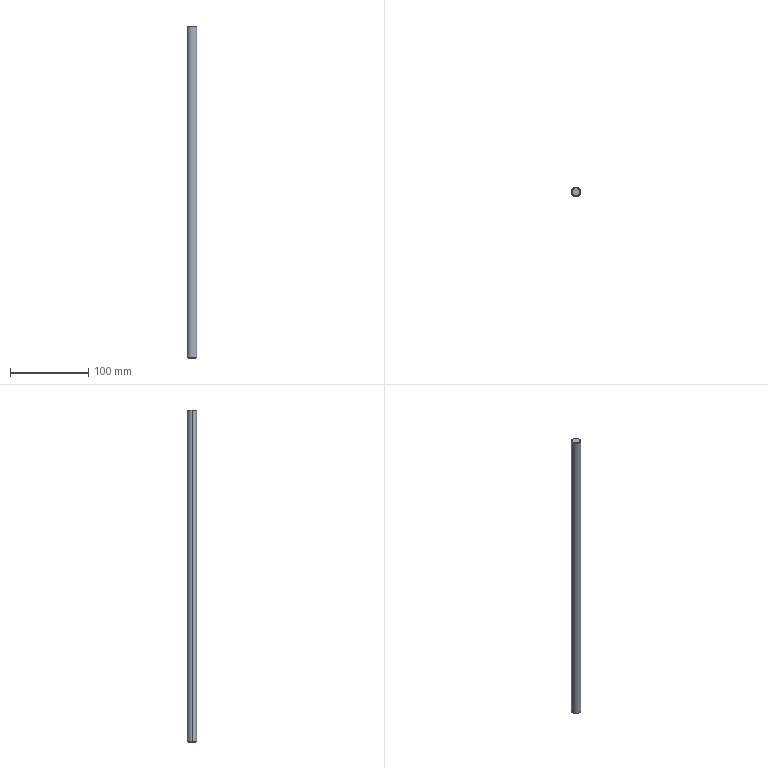Component | SolidWorks | 50-2 | 1 solid | 8 faces | box 12 x 12 x 425 mm | volume 48031 mm3 | cone 4 | cylinder 2 | plane 2 | commonest cylinder face diameters 12 x2
build123d program:
from build123d import *

# Parameters (mm, degrees)
SKETCH1_W     = 425
SKETCH1_H     = 6
CHAMFER1_SIZE = 1


with BuildPart() as part:
    # Sketch1 → Revolve1 (revolve)
    with BuildSketch(Plane.XY, mode=Mode.PRIVATE) as revolve1_sk:
        with Locations((212.5, 3)):
            Rectangle(SKETCH1_W, SKETCH1_H)
    revolve(revolve1_sk.sketch.rotate(Axis((0, 0, 0), (1, 0, 0)), 90), axis=Axis((0, 0, 0), (1, 0, 0)))

    # Chamfer1
    chamfer1_edges = [part.edges().sort_by_distance(p)[0] for p in [
        (425, 0, -6),
        (0, 0, -6),
    ]]
    chamfer(chamfer1_edges, length=CHAMFER1_SIZE)


solid = part.part

# Placed as in the assembly
solid = solid.moved(Location((0, -38, 427.5), (0, 90, 0)))
STEP:
#1=COLOUR_RGB('',0.7922,0.8196,0.9333);
#2=FILL_AREA_STYLE_COLOUR('',#1);
#3=FILL_AREA_STYLE('',(#2));
#4=SURFACE_STYLE_FILL_AREA(#3);
#5=SURFACE_SIDE_STYLE('',(#4));
#6=SURFACE_STYLE_USAGE(.BOTH.,#5);
#7=PRESENTATION_STYLE_ASSIGNMENT((#6));
#8=CARTESIAN_POINT('',(0.1969,-1.496,16.831));
#9=VERTEX_POINT('',#8);
#10=CARTESIAN_POINT('',(-0.1969,-1.496,16.831));
#11=VERTEX_POINT('',#10);
#12=CARTESIAN_POINT('',(-0.,-1.496,16.831));
#13=DIRECTION('',(0.,0.,1.));
#14=DIRECTION('',(-1.,0.,0.));
#15=AXIS2_PLACEMENT_3D('',#12,#13,#14);
#16=CIRCLE('',#15,0.1969);
#17=EDGE_CURVE('',#9,#11,#16,.T.);
#18=ORIENTED_EDGE('',*,*,#17,.F.);
#19=CARTESIAN_POINT('',(0.2362,-1.496,16.791));
#20=VERTEX_POINT('',#19);
#21=CARTESIAN_POINT('',(0.1969,-1.496,16.831));
#22=DIRECTION('',(0.7071,-0.,-0.7071));
#23=VECTOR('',#22,39.37);
#24=LINE('',#21,#23);
#25=EDGE_CURVE('',#9,#20,#24,.T.);
#26=ORIENTED_EDGE('',*,*,#25,.T.);
#27=CARTESIAN_POINT('',(-0.2362,-1.496,16.791));
#28=VERTEX_POINT('',#27);
#29=CARTESIAN_POINT('',(-0.,-1.496,16.791));
#30=DIRECTION('',(-0.,-0.,-1.));
#31=DIRECTION('',(-1.,0.,0.));
#32=AXIS2_PLACEMENT_3D('',#29,#30,#31);
#33=CIRCLE('',#32,0.2362);
#34=EDGE_CURVE('',#28,#20,#33,.T.);
#35=ORIENTED_EDGE('',*,*,#34,.F.);
#36=CARTESIAN_POINT('',(-0.1969,-1.496,16.831));
#37=DIRECTION('',(-0.7071,-0.,-0.7071));
#38=VECTOR('',#37,39.37);
#39=LINE('',#36,#38);
#40=EDGE_CURVE('',#11,#28,#39,.T.);
#41=ORIENTED_EDGE('',*,*,#40,.F.);
#42=EDGE_LOOP('',(#18,#26,#35,#41));
#43=FACE_OUTER_BOUND('',#42,.T.);
#44=CARTESIAN_POINT('',(-0.,-1.496,16.831));
#45=DIRECTION('',(-0.,-0.,-1.));
#46=DIRECTION('',(-1.,0.,0.));
#47=AXIS2_PLACEMENT_3D('',#44,#45,#46);
#48=CONICAL_SURFACE('',#47,0.1969,0.7854);
#49=ADVANCED_FACE('',(#43),#48,.T.);
#50=CARTESIAN_POINT('',(-0.1969,-1.496,0.09843));
#51=VERTEX_POINT('',#50);
#52=CARTESIAN_POINT('',(0.1969,-1.496,0.09843));
#53=VERTEX_POINT('',#52);
#54=CARTESIAN_POINT('',(-0.,-1.496,0.09843));
#55=DIRECTION('',(-0.,-0.,-1.));
#56=DIRECTION('',(1.,0.,0.));
#57=AXIS2_PLACEMENT_3D('',#54,#55,#56);
#58=CIRCLE('',#57,0.1969);
#59=EDGE_CURVE('',#51,#53,#58,.T.);
#60=ORIENTED_EDGE('',*,*,#59,.F.);
#61=CARTESIAN_POINT('',(-0.2362,-1.496,0.1378));
#62=VERTEX_POINT('',#61);
#63=CARTESIAN_POINT('',(-0.2362,-1.496,0.1378));
#64=DIRECTION('',(-0.7071,0.,0.7071));
#65=VECTOR('',#64,39.37);
#66=LINE('',#63,#65);
#67=EDGE_CURVE('',#51,#62,#66,.T.);
#68=ORIENTED_EDGE('',*,*,#67,.T.);
#69=CARTESIAN_POINT('',(0.2362,-1.496,0.1378));
#70=VERTEX_POINT('',#69);
#71=CARTESIAN_POINT('',(-0.,-1.496,0.1378));
#72=DIRECTION('',(0.,0.,1.));
#73=DIRECTION('',(1.,0.,0.));
#74=AXIS2_PLACEMENT_3D('',#71,#72,#73);
#75=CIRCLE('',#74,0.2362);
#76=EDGE_CURVE('',#70,#62,#75,.T.);
#77=ORIENTED_EDGE('',*,*,#76,.F.);
#78=CARTESIAN_POINT('',(0.2362,-1.496,0.1378));
#79=DIRECTION('',(0.7071,0.,0.7071));
#80=VECTOR('',#79,39.37);
#81=LINE('',#78,#80);
#82=EDGE_CURVE('',#53,#70,#81,.T.);
#83=ORIENTED_EDGE('',*,*,#82,.F.);
#84=EDGE_LOOP('',(#60,#68,#77,#83));
#85=FACE_OUTER_BOUND('',#84,.T.);
#86=CARTESIAN_POINT('',(-0.,-1.496,0.1378));
#87=DIRECTION('',(0.,0.,1.));
#88=DIRECTION('',(1.,0.,0.));
#89=AXIS2_PLACEMENT_3D('',#86,#87,#88);
#90=CONICAL_SURFACE('',#89,0.2362,0.7854);
#91=ADVANCED_FACE('',(#85),#90,.T.);
#92=ORIENTED_EDGE('',*,*,#76,.T.);
#93=CARTESIAN_POINT('',(-0.2362,-1.496,16.831));
#94=DIRECTION('',(0.,0.,1.));
#95=VECTOR('',#94,39.37);
#96=LINE('',#93,#95);
#97=EDGE_CURVE('',#62,#28,#96,.T.);
#98=ORIENTED_EDGE('',*,*,#97,.T.);
#99=ORIENTED_EDGE('',*,*,#34,.T.);
#100=CARTESIAN_POINT('',(0.2362,-1.496,16.831));
#101=DIRECTION('',(0.,0.,1.));
#102=VECTOR('',#101,39.37);
#103=LINE('',#100,#102);
#104=EDGE_CURVE('',#70,#20,#103,.T.);
#105=ORIENTED_EDGE('',*,*,#104,.F.);
#106=EDGE_LOOP('',(#92,#98,#99,#105));
#107=FACE_OUTER_BOUND('',#106,.T.);
#108=CARTESIAN_POINT('',(-0.,-1.496,16.831));
#109=DIRECTION('',(0.,0.,1.));
#110=DIRECTION('',(1.,0.,0.));
#111=AXIS2_PLACEMENT_3D('',#108,#109,#110);
#112=CYLINDRICAL_SURFACE('',#111,0.2362);
#113=ADVANCED_FACE('',(#107),#112,.T.);
#114=CARTESIAN_POINT('',(-0.,-1.496,16.831));
#115=DIRECTION('',(0.,0.,1.));
#116=DIRECTION('',(-1.,0.,0.));
#117=AXIS2_PLACEMENT_3D('',#114,#115,#116);
#118=CIRCLE('',#117,0.1969);
#119=EDGE_CURVE('',#11,#9,#118,.T.);
#120=ORIENTED_EDGE('',*,*,#119,.T.);
#121=ORIENTED_EDGE('',*,*,#17,.T.);
#122=EDGE_LOOP('',(#120,#121));
#123=FACE_OUTER_BOUND('',#122,.T.);
#124=CARTESIAN_POINT('',(-0.,-1.496,16.831));
#125=DIRECTION('',(-0.,-0.,-1.));
#126=DIRECTION('',(-1.,0.,-0.));
#127=AXIS2_PLACEMENT_3D('',#124,#125,#126);
#128=PLANE('',#127);
#129=ADVANCED_FACE('',(#123),#128,.F.);
#130=ORIENTED_EDGE('',*,*,#97,.F.);
#131=CARTESIAN_POINT('',(-0.,-1.496,0.1378));
#132=DIRECTION('',(0.,0.,1.));
#133=DIRECTION('',(1.,0.,0.));
#134=AXIS2_PLACEMENT_3D('',#131,#132,#133);
#135=CIRCLE('',#134,0.2362);
#136=EDGE_CURVE('',#62,#70,#135,.T.);
#137=ORIENTED_EDGE('',*,*,#136,.T.);
#138=ORIENTED_EDGE('',*,*,#104,.T.);
#139=CARTESIAN_POINT('',(-0.,-1.496,16.791));
#140=DIRECTION('',(-0.,-0.,-1.));
#141=DIRECTION('',(-1.,0.,0.));
#142=AXIS2_PLACEMENT_3D('',#139,#140,#141);
#143=CIRCLE('',#142,0.2362);
#144=EDGE_CURVE('',#20,#28,#143,.T.);
#145=ORIENTED_EDGE('',*,*,#144,.T.);
#146=EDGE_LOOP('',(#130,#137,#138,#145));
#147=FACE_OUTER_BOUND('',#146,.T.);
#148=CARTESIAN_POINT('',(-0.,-1.496,16.831));
#149=DIRECTION('',(0.,0.,1.));
#150=DIRECTION('',(1.,0.,0.));
#151=AXIS2_PLACEMENT_3D('',#148,#149,#150);
#152=CYLINDRICAL_SURFACE('',#151,0.2362);
#153=ADVANCED_FACE('',(#147),#152,.T.);
#154=CARTESIAN_POINT('',(-0.,-1.496,0.09843));
#155=DIRECTION('',(-0.,-0.,-1.));
#156=DIRECTION('',(1.,0.,0.));
#157=AXIS2_PLACEMENT_3D('',#154,#155,#156);
#158=CIRCLE('',#157,0.1969);
#159=EDGE_CURVE('',#53,#51,#158,.T.);
#160=ORIENTED_EDGE('',*,*,#159,.T.);
#161=ORIENTED_EDGE('',*,*,#59,.T.);
#162=EDGE_LOOP('',(#160,#161));
#163=FACE_OUTER_BOUND('',#162,.T.);
#164=CARTESIAN_POINT('',(-0.,-1.496,0.09843));
#165=DIRECTION('',(0.,0.,1.));
#166=DIRECTION('',(1.,-0.,0.));
#167=AXIS2_PLACEMENT_3D('',#164,#165,#166);
#168=PLANE('',#167);
#169=ADVANCED_FACE('',(#163),#168,.F.);
#170=ORIENTED_EDGE('',*,*,#67,.F.);
#171=ORIENTED_EDGE('',*,*,#159,.F.);
#172=ORIENTED_EDGE('',*,*,#82,.T.);
#173=ORIENTED_EDGE('',*,*,#136,.F.);
#174=EDGE_LOOP('',(#170,#171,#172,#173));
#175=FACE_OUTER_BOUND('',#174,.T.);
#176=CARTESIAN_POINT('',(-0.,-1.496,0.1378));
#177=DIRECTION('',(0.,0.,1.));
#178=DIRECTION('',(1.,0.,0.));
#179=AXIS2_PLACEMENT_3D('',#176,#177,#178);
#180=CONICAL_SURFACE('',#179,0.2362,0.7854);
#181=ADVANCED_FACE('',(#175),#180,.T.);
#182=ORIENTED_EDGE('',*,*,#25,.F.);
#183=ORIENTED_EDGE('',*,*,#119,.F.);
#184=ORIENTED_EDGE('',*,*,#40,.T.);
#185=ORIENTED_EDGE('',*,*,#144,.F.);
#186=EDGE_LOOP('',(#182,#183,#184,#185));
#187=FACE_OUTER_BOUND('',#186,.T.);
#188=CARTESIAN_POINT('',(-0.,-1.496,16.831));
#189=DIRECTION('',(-0.,-0.,-1.));
#190=DIRECTION('',(-1.,0.,0.));
#191=AXIS2_PLACEMENT_3D('',#188,#189,#190);
#192=CONICAL_SURFACE('',#191,0.1969,0.7854);
#193=ADVANCED_FACE('',(#187),#192,.T.);
#194=CLOSED_SHELL('',(#49,#91,#113,#129,#153,#169,#181,#193));
#195=MANIFOLD_SOLID_BREP('',#194);
#196=STYLED_ITEM('',(#7),#195);
#197=PRESENTATION_LAYER_ASSIGNMENT('','',(#196));
#198=(LENGTH_UNIT()NAMED_UNIT(*)SI_UNIT($,.METRE.));
#199=LENGTH_MEASURE_WITH_UNIT(LENGTH_MEASURE(0.0254),#198);
#200=DIMENSIONAL_EXPONENTS(1.,0.,0.,0.,0.,0.,0.);
#201=(CONVERSION_BASED_UNIT('',#199)LENGTH_UNIT()NAMED_UNIT(#200));
#202=UNCERTAINTY_MEASURE_WITH_UNIT(LENGTH_MEASURE(0.00001),#201,'','');
#203=(NAMED_UNIT(*)PLANE_ANGLE_UNIT()SI_UNIT($,.RADIAN.));
#204=(NAMED_UNIT(*)SI_UNIT($,.STERADIAN.)SOLID_ANGLE_UNIT());
#205=(GEOMETRIC_REPRESENTATION_CONTEXT(3)GLOBAL_UNCERTAINTY_ASSIGNED_CONTEXT((#202))GLOBAL_UNIT_ASSIGNED_CONTEXT((#201,#203,#204))REPRESENTATION_CONTEXT('',''));
#206=MECHANICAL_DESIGN_GEOMETRIC_PRESENTATION_REPRESENTATION('',(#196),#205);
#207=CARTESIAN_POINT('',(0.,0.,0.));
#208=DIRECTION('',(0.,0.,1.));
#209=DIRECTION('',(1.,0.,0.));
#210=AXIS2_PLACEMENT_3D('',#207,#208,#209);
#211=(LENGTH_UNIT()NAMED_UNIT(*)SI_UNIT($,.METRE.));
#212=LENGTH_MEASURE_WITH_UNIT(LENGTH_MEASURE(0.0254),#211);
#213=DIMENSIONAL_EXPONENTS(1.,0.,0.,0.,0.,0.,0.);
#214=(CONVERSION_BASED_UNIT('',#212)LENGTH_UNIT()NAMED_UNIT(#213));
#215=UNCERTAINTY_MEASURE_WITH_UNIT(LENGTH_MEASURE(0.00001),#214,'','');
#216=(NAMED_UNIT(*)PLANE_ANGLE_UNIT()SI_UNIT($,.RADIAN.));
#217=(NAMED_UNIT(*)SI_UNIT($,.STERADIAN.)SOLID_ANGLE_UNIT());
#218=(GEOMETRIC_REPRESENTATION_CONTEXT(3)GLOBAL_UNCERTAINTY_ASSIGNED_CONTEXT((#215))GLOBAL_UNIT_ASSIGNED_CONTEXT((#214,#216,#217))REPRESENTATION_CONTEXT('',''));
#219=ADVANCED_BREP_SHAPE_REPRESENTATION('',(#195,#210),#218);